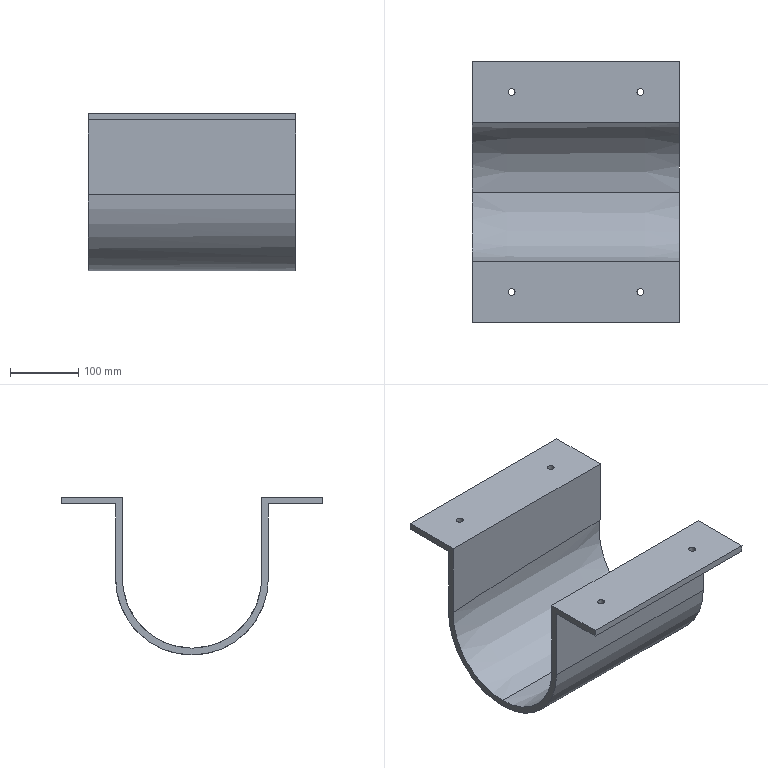Component | SolidWorks | Accessory1-3 | 1 solid | 31 faces | box 304.83 x 384.16 x 231.67 mm | volume 2139053 mm3 | plane 12 | cone 10 | cylinder 9 | commonest cylinder face diameters 10 x8 224.162 x1
STEP:
#1=COLOUR_RGB('',0.7922,0.8196,0.9333);
#2=FILL_AREA_STYLE_COLOUR('',#1);
#3=FILL_AREA_STYLE('',(#2));
#4=SURFACE_STYLE_FILL_AREA(#3);
#5=SURFACE_SIDE_STYLE('',(#4));
#6=SURFACE_STYLE_USAGE(.BOTH.,#5);
#7=PRESENTATION_STYLE_ASSIGNMENT((#6));
#8=CARTESIAN_POINT('',(-60.943,275.591,-4.023));
#9=VERTEX_POINT('',#8);
#10=CARTESIAN_POINT('',(-60.943,279.609,0.1806));
#11=VERTEX_POINT('',#10);
#12=CARTESIAN_POINT('',(-60.943,275.591,0.));
#13=DIRECTION('',(1.,-0.,-0.));
#14=DIRECTION('',(0.,0.,1.));
#15=AXIS2_PLACEMENT_3D('',#12,#13,#14);
#16=CIRCLE('',#15,4.023);
#17=EDGE_CURVE('',#9,#11,#16,.T.);
#18=ORIENTED_EDGE('',*,*,#17,.F.);
#19=CARTESIAN_POINT('',(-48.98,275.591,-4.088));
#20=VERTEX_POINT('',#19);
#21=CARTESIAN_POINT('',(-48.738,275.591,-4.089));
#22=DIRECTION('',(1.,-0.,-0.005413));
#23=VECTOR('',#22,39.37);
#24=LINE('',#21,#23);
#25=EDGE_CURVE('',#9,#20,#24,.T.);
#26=ORIENTED_EDGE('',*,*,#25,.T.);
#27=CARTESIAN_POINT('',(-48.959,279.609,0.7475));
#28=VERTEX_POINT('',#27);
#29=CARTESIAN_POINT('',(-48.98,275.591,-4.088));
#30=CARTESIAN_POINT('',(-48.98,278.35,-4.088));
#31=CARTESIAN_POINT('',(-48.971,280.114,-1.966));
#32=CARTESIAN_POINT('',(-48.959,279.609,0.7475));
#33=(BOUNDED_CURVE()B_SPLINE_CURVE(3,(#29,#30,#31,#32),.UNSPECIFIED.,.F.,.F.)B_SPLINE_CURVE_WITH_KNOTS((4,4),(3.142,4.896),.UNSPECIFIED.)CURVE()GEOMETRIC_REPRESENTATION_ITEM()RATIONAL_B_SPLINE_CURVE((1.,0.7595,0.7595,1.))REPRESENTATION_ITEM(''));
#34=EDGE_CURVE('',#20,#28,#33,.T.);
#35=ORIENTED_EDGE('',*,*,#34,.T.);
#36=CARTESIAN_POINT('',(-60.943,279.609,0.1806));
#37=CARTESIAN_POINT('',(-60.819,279.609,0.1956));
#38=CARTESIAN_POINT('',(-60.695,279.609,0.2088));
#39=CARTESIAN_POINT('',(-60.446,279.609,0.2333));
#40=CARTESIAN_POINT('',(-60.321,279.609,0.2446));
#41=CARTESIAN_POINT('',(-59.948,279.609,0.2765));
#42=CARTESIAN_POINT('',(-59.698,279.609,0.2953));
#43=CARTESIAN_POINT('',(-59.2,279.609,0.3301));
#44=CARTESIAN_POINT('',(-58.95,279.609,0.3461));
#45=CARTESIAN_POINT('',(-58.451,279.609,0.3763));
#46=CARTESIAN_POINT('',(-58.201,279.609,0.3904));
#47=CARTESIAN_POINT('',(-57.452,279.609,0.431));
#48=CARTESIAN_POINT('',(-56.953,279.609,0.4554));
#49=CARTESIAN_POINT('',(-55.954,279.609,0.5012));
#50=CARTESIAN_POINT('',(-55.455,279.609,0.5225));
#51=CARTESIAN_POINT('',(-53.956,279.609,0.5831));
#52=CARTESIAN_POINT('',(-52.957,279.609,0.6192));
#53=CARTESIAN_POINT('',(-50.958,279.609,0.6867));
#54=CARTESIAN_POINT('',(-49.958,279.609,0.7179));
#55=CARTESIAN_POINT('',(-48.959,279.609,0.7475));
#56=B_SPLINE_CURVE_WITH_KNOTS('',3,(#36,#37,#38,#39,#40,#41,#42,#43,#44,#45,#46,#47,#48,#49,#50,#51,#52,#53,#54,#55),.UNSPECIFIED.,.F.,.F.,(4,2,2,2,2,2,2,2,2,4),(0.02686,0.03643,0.046,0.06513,0.08427,0.1034,0.1417,0.18,0.2565,0.3331),.UNSPECIFIED.);
#57=EDGE_CURVE('',#11,#28,#56,.T.);
#58=ORIENTED_EDGE('',*,*,#57,.F.);
#59=EDGE_LOOP('',(#18,#26,#35,#58));
#60=FACE_OUTER_BOUND('',#59,.T.);
#61=CARTESIAN_POINT('',(-48.738,275.591,0.));
#62=DIRECTION('',(1.,-0.,-0.));
#63=DIRECTION('',(0.,0.,-1.));
#64=AXIS2_PLACEMENT_3D('',#61,#62,#63);
#65=CONICAL_SURFACE('',#64,4.089,0.005413);
#66=ADVANCED_FACE('',(#60),#65,.F.);
#67=CARTESIAN_POINT('',(-51.029,281.365,4.334));
#68=VERTEX_POINT('',#67);
#69=CARTESIAN_POINT('',(-51.422,281.365,4.334));
#70=VERTEX_POINT('',#69);
#71=CARTESIAN_POINT('',(-51.225,281.365,4.334));
#72=DIRECTION('',(-0.,0.,-1.));
#73=DIRECTION('',(-1.,0.,0.));
#74=AXIS2_PLACEMENT_3D('',#71,#72,#73);
#75=CIRCLE('',#74,0.1969);
#76=EDGE_CURVE('',#68,#70,#75,.T.);
#77=ORIENTED_EDGE('',*,*,#76,.F.);
#78=CARTESIAN_POINT('',(-51.009,281.365,4.315));
#79=VERTEX_POINT('',#78);
#80=CARTESIAN_POINT('',(-51.029,281.365,4.334));
#81=DIRECTION('',(0.7071,0.,-0.7071));
#82=VECTOR('',#81,39.37);
#83=LINE('',#80,#82);
#84=EDGE_CURVE('',#68,#79,#83,.T.);
#85=ORIENTED_EDGE('',*,*,#84,.T.);
#86=CARTESIAN_POINT('',(-51.442,281.365,4.315));
#87=VERTEX_POINT('',#86);
#88=CARTESIAN_POINT('',(-51.225,281.365,4.315));
#89=DIRECTION('',(0.,-0.,1.));
#90=DIRECTION('',(-1.,0.,0.));
#91=AXIS2_PLACEMENT_3D('',#88,#89,#90);
#92=CIRCLE('',#91,0.2165);
#93=EDGE_CURVE('',#87,#79,#92,.T.);
#94=ORIENTED_EDGE('',*,*,#93,.F.);
#95=CARTESIAN_POINT('',(-51.422,281.365,4.334));
#96=DIRECTION('',(-0.7071,0.,-0.7071));
#97=VECTOR('',#96,39.37);
#98=LINE('',#95,#97);
#99=EDGE_CURVE('',#70,#87,#98,.T.);
#100=ORIENTED_EDGE('',*,*,#99,.F.);
#101=EDGE_LOOP('',(#77,#85,#94,#100));
#102=FACE_OUTER_BOUND('',#101,.T.);
#103=CARTESIAN_POINT('',(-51.225,281.365,4.334));
#104=DIRECTION('',(-0.,0.,-1.));
#105=DIRECTION('',(-1.,0.,0.));
#106=AXIS2_PLACEMENT_3D('',#103,#104,#105);
#107=CONICAL_SURFACE('',#106,0.1969,0.7854);
#108=ADVANCED_FACE('',(#102),#107,.F.);
#109=CARTESIAN_POINT('',(-58.464,281.365,4.334));
#110=VERTEX_POINT('',#109);
#111=CARTESIAN_POINT('',(-58.858,281.365,4.334));
#112=VERTEX_POINT('',#111);
#113=CARTESIAN_POINT('',(-58.661,281.365,4.334));
#114=DIRECTION('',(-0.,0.,-1.));
#115=DIRECTION('',(-1.,0.,0.));
#116=AXIS2_PLACEMENT_3D('',#113,#114,#115);
#117=CIRCLE('',#116,0.1969);
#118=EDGE_CURVE('',#110,#112,#117,.T.);
#119=ORIENTED_EDGE('',*,*,#118,.F.);
#120=CARTESIAN_POINT('',(-58.445,281.365,4.315));
#121=VERTEX_POINT('',#120);
#122=CARTESIAN_POINT('',(-58.464,281.365,4.334));
#123=DIRECTION('',(0.7071,0.,-0.7071));
#124=VECTOR('',#123,39.37);
#125=LINE('',#122,#124);
#126=EDGE_CURVE('',#110,#121,#125,.T.);
#127=ORIENTED_EDGE('',*,*,#126,.T.);
#128=CARTESIAN_POINT('',(-58.878,281.365,4.315));
#129=VERTEX_POINT('',#128);
#130=CARTESIAN_POINT('',(-58.661,281.365,4.315));
#131=DIRECTION('',(0.,-0.,1.));
#132=DIRECTION('',(-1.,0.,0.));
#133=AXIS2_PLACEMENT_3D('',#130,#131,#132);
#134=CIRCLE('',#133,0.2165);
#135=EDGE_CURVE('',#129,#121,#134,.T.);
#136=ORIENTED_EDGE('',*,*,#135,.F.);
#137=CARTESIAN_POINT('',(-58.858,281.365,4.334));
#138=DIRECTION('',(-0.7071,0.,-0.7071));
#139=VECTOR('',#138,39.37);
#140=LINE('',#137,#139);
#141=EDGE_CURVE('',#112,#129,#140,.T.);
#142=ORIENTED_EDGE('',*,*,#141,.F.);
#143=EDGE_LOOP('',(#119,#127,#136,#142));
#144=FACE_OUTER_BOUND('',#143,.T.);
#145=CARTESIAN_POINT('',(-58.661,281.365,4.334));
#146=DIRECTION('',(-0.,0.,-1.));
#147=DIRECTION('',(-1.,0.,0.));
#148=AXIS2_PLACEMENT_3D('',#145,#146,#147);
#149=CONICAL_SURFACE('',#148,0.1969,0.7854);
#150=ADVANCED_FACE('',(#144),#149,.F.);
#151=CARTESIAN_POINT('',(-51.029,269.816,4.334));
#152=VERTEX_POINT('',#151);
#153=CARTESIAN_POINT('',(-51.422,269.816,4.334));
#154=VERTEX_POINT('',#153);
#155=CARTESIAN_POINT('',(-51.225,269.816,4.334));
#156=DIRECTION('',(-0.,0.,-1.));
#157=DIRECTION('',(-1.,0.,0.));
#158=AXIS2_PLACEMENT_3D('',#155,#156,#157);
#159=CIRCLE('',#158,0.1969);
#160=EDGE_CURVE('',#152,#154,#159,.T.);
#161=ORIENTED_EDGE('',*,*,#160,.F.);
#162=CARTESIAN_POINT('',(-51.009,269.816,4.315));
#163=VERTEX_POINT('',#162);
#164=CARTESIAN_POINT('',(-51.029,269.816,4.334));
#165=DIRECTION('',(0.7071,0.,-0.7071));
#166=VECTOR('',#165,39.37);
#167=LINE('',#164,#166);
#168=EDGE_CURVE('',#152,#163,#167,.T.);
#169=ORIENTED_EDGE('',*,*,#168,.T.);
#170=CARTESIAN_POINT('',(-51.442,269.816,4.315));
#171=VERTEX_POINT('',#170);
#172=CARTESIAN_POINT('',(-51.225,269.816,4.315));
#173=DIRECTION('',(0.,0.,1.));
#174=DIRECTION('',(0.,-1.,0.));
#175=AXIS2_PLACEMENT_3D('',#172,#173,#174);
#176=CIRCLE('',#175,0.2165);
#177=EDGE_CURVE('',#171,#163,#176,.T.);
#178=ORIENTED_EDGE('',*,*,#177,.F.);
#179=CARTESIAN_POINT('',(-51.422,269.816,4.334));
#180=DIRECTION('',(-0.7071,0.,-0.7071));
#181=VECTOR('',#180,39.37);
#182=LINE('',#179,#181);
#183=EDGE_CURVE('',#154,#171,#182,.T.);
#184=ORIENTED_EDGE('',*,*,#183,.F.);
#185=EDGE_LOOP('',(#161,#169,#178,#184));
#186=FACE_OUTER_BOUND('',#185,.T.);
#187=CARTESIAN_POINT('',(-51.225,269.816,4.334));
#188=DIRECTION('',(-0.,0.,-1.));
#189=DIRECTION('',(-1.,0.,0.));
#190=AXIS2_PLACEMENT_3D('',#187,#188,#189);
#191=CONICAL_SURFACE('',#190,0.1969,0.7854);
#192=ADVANCED_FACE('',(#186),#191,.F.);
#193=CARTESIAN_POINT('',(-58.464,269.816,4.334));
#194=VERTEX_POINT('',#193);
#195=CARTESIAN_POINT('',(-58.858,269.816,4.334));
#196=VERTEX_POINT('',#195);
#197=CARTESIAN_POINT('',(-58.661,269.816,4.334));
#198=DIRECTION('',(-0.,0.,-1.));
#199=DIRECTION('',(-1.,0.,0.));
#200=AXIS2_PLACEMENT_3D('',#197,#198,#199);
#201=CIRCLE('',#200,0.1969);
#202=EDGE_CURVE('',#194,#196,#201,.T.);
#203=ORIENTED_EDGE('',*,*,#202,.F.);
#204=CARTESIAN_POINT('',(-58.445,269.816,4.315));
#205=VERTEX_POINT('',#204);
#206=CARTESIAN_POINT('',(-58.464,269.816,4.334));
#207=DIRECTION('',(0.7071,0.,-0.7071));
#208=VECTOR('',#207,39.37);
#209=LINE('',#206,#208);
#210=EDGE_CURVE('',#194,#205,#209,.T.);
#211=ORIENTED_EDGE('',*,*,#210,.T.);
#212=CARTESIAN_POINT('',(-58.878,269.816,4.315));
#213=VERTEX_POINT('',#212);
#214=CARTESIAN_POINT('',(-58.661,269.816,4.315));
#215=DIRECTION('',(0.,0.,1.));
#216=DIRECTION('',(0.,-1.,0.));
#217=AXIS2_PLACEMENT_3D('',#214,#215,#216);
#218=CIRCLE('',#217,0.2165);
#219=EDGE_CURVE('',#213,#205,#218,.T.);
#220=ORIENTED_EDGE('',*,*,#219,.F.);
#221=CARTESIAN_POINT('',(-58.858,269.816,4.334));
#222=DIRECTION('',(-0.7071,0.,-0.7071));
#223=VECTOR('',#222,39.37);
#224=LINE('',#221,#223);
#225=EDGE_CURVE('',#196,#213,#224,.T.);
#226=ORIENTED_EDGE('',*,*,#225,.F.);
#227=EDGE_LOOP('',(#203,#211,#220,#226));
#228=FACE_OUTER_BOUND('',#227,.T.);
#229=CARTESIAN_POINT('',(-58.661,269.816,4.334));
#230=DIRECTION('',(-0.,0.,-1.));
#231=DIRECTION('',(-1.,0.,0.));
#232=AXIS2_PLACEMENT_3D('',#229,#230,#231);
#233=CONICAL_SURFACE('',#232,0.1969,0.7854);
#234=ADVANCED_FACE('',(#228),#233,.F.);
#235=CARTESIAN_POINT('',(-58.858,281.365,4.708));
#236=VERTEX_POINT('',#235);
#237=CARTESIAN_POINT('',(-58.464,281.365,4.708));
#238=VERTEX_POINT('',#237);
#239=CARTESIAN_POINT('',(-58.661,281.365,4.708));
#240=DIRECTION('',(0.,-0.,1.));
#241=DIRECTION('',(1.,0.,0.));
#242=AXIS2_PLACEMENT_3D('',#239,#240,#241);
#243=CIRCLE('',#242,0.1969);
#244=EDGE_CURVE('',#236,#238,#243,.T.);
#245=ORIENTED_EDGE('',*,*,#244,.T.);
#246=CARTESIAN_POINT('',(-58.464,281.365,18.882));
#247=DIRECTION('',(-0.,0.,-1.));
#248=VECTOR('',#247,39.37);
#249=LINE('',#246,#248);
#250=EDGE_CURVE('',#238,#110,#249,.T.);
#251=ORIENTED_EDGE('',*,*,#250,.T.);
#252=ORIENTED_EDGE('',*,*,#118,.T.);
#253=CARTESIAN_POINT('',(-58.858,281.365,18.882));
#254=DIRECTION('',(-0.,0.,-1.));
#255=VECTOR('',#254,39.37);
#256=LINE('',#253,#255);
#257=EDGE_CURVE('',#236,#112,#256,.T.);
#258=ORIENTED_EDGE('',*,*,#257,.F.);
#259=EDGE_LOOP('',(#245,#251,#252,#258));
#260=FACE_OUTER_BOUND('',#259,.T.);
#261=CARTESIAN_POINT('',(-58.661,281.365,18.882));
#262=DIRECTION('',(-0.,0.,-1.));
#263=DIRECTION('',(-1.,0.,0.));
#264=AXIS2_PLACEMENT_3D('',#261,#262,#263);
#265=CYLINDRICAL_SURFACE('',#264,0.1969);
#266=ADVANCED_FACE('',(#260),#265,.F.);
#267=CARTESIAN_POINT('',(-51.422,281.365,4.708));
#268=VERTEX_POINT('',#267);
#269=CARTESIAN_POINT('',(-51.029,281.365,4.708));
#270=VERTEX_POINT('',#269);
#271=CARTESIAN_POINT('',(-51.225,281.365,4.708));
#272=DIRECTION('',(0.,-0.,1.));
#273=DIRECTION('',(1.,0.,0.));
#274=AXIS2_PLACEMENT_3D('',#271,#272,#273);
#275=CIRCLE('',#274,0.1969);
#276=EDGE_CURVE('',#268,#270,#275,.T.);
#277=ORIENTED_EDGE('',*,*,#276,.T.);
#278=CARTESIAN_POINT('',(-51.029,281.365,18.882));
#279=DIRECTION('',(-0.,0.,-1.));
#280=VECTOR('',#279,39.37);
#281=LINE('',#278,#280);
#282=EDGE_CURVE('',#270,#68,#281,.T.);
#283=ORIENTED_EDGE('',*,*,#282,.T.);
#284=ORIENTED_EDGE('',*,*,#76,.T.);
#285=CARTESIAN_POINT('',(-51.422,281.365,18.882));
#286=DIRECTION('',(-0.,0.,-1.));
#287=VECTOR('',#286,39.37);
#288=LINE('',#285,#287);
#289=EDGE_CURVE('',#268,#70,#288,.T.);
#290=ORIENTED_EDGE('',*,*,#289,.F.);
#291=EDGE_LOOP('',(#277,#283,#284,#290));
#292=FACE_OUTER_BOUND('',#291,.T.);
#293=CARTESIAN_POINT('',(-51.225,281.365,18.882));
#294=DIRECTION('',(-0.,0.,-1.));
#295=DIRECTION('',(-1.,0.,0.));
#296=AXIS2_PLACEMENT_3D('',#293,#294,#295);
#297=CYLINDRICAL_SURFACE('',#296,0.1969);
#298=ADVANCED_FACE('',(#292),#297,.F.);
#299=CARTESIAN_POINT('',(-51.422,269.816,4.708));
#300=VERTEX_POINT('',#299);
#301=CARTESIAN_POINT('',(-51.029,269.816,4.708));
#302=VERTEX_POINT('',#301);
#303=CARTESIAN_POINT('',(-51.225,269.816,4.708));
#304=DIRECTION('',(0.,-0.,1.));
#305=DIRECTION('',(1.,0.,0.));
#306=AXIS2_PLACEMENT_3D('',#303,#304,#305);
#307=CIRCLE('',#306,0.1969);
#308=EDGE_CURVE('',#300,#302,#307,.T.);
#309=ORIENTED_EDGE('',*,*,#308,.T.);
#310=CARTESIAN_POINT('',(-51.029,269.816,18.882));
#311=DIRECTION('',(-0.,0.,-1.));
#312=VECTOR('',#311,39.37);
#313=LINE('',#310,#312);
#314=EDGE_CURVE('',#302,#152,#313,.T.);
#315=ORIENTED_EDGE('',*,*,#314,.T.);
#316=ORIENTED_EDGE('',*,*,#160,.T.);
#317=CARTESIAN_POINT('',(-51.422,269.816,18.882));
#318=DIRECTION('',(-0.,0.,-1.));
#319=VECTOR('',#318,39.37);
#320=LINE('',#317,#319);
#321=EDGE_CURVE('',#300,#154,#320,.T.);
#322=ORIENTED_EDGE('',*,*,#321,.F.);
#323=EDGE_LOOP('',(#309,#315,#316,#322));
#324=FACE_OUTER_BOUND('',#323,.T.);
#325=CARTESIAN_POINT('',(-51.225,269.816,18.882));
#326=DIRECTION('',(-0.,0.,-1.));
#327=DIRECTION('',(-1.,0.,0.));
#328=AXIS2_PLACEMENT_3D('',#325,#326,#327);
#329=CYLINDRICAL_SURFACE('',#328,0.1969);
#330=ADVANCED_FACE('',(#324),#329,.F.);
#331=CARTESIAN_POINT('',(-58.858,269.816,4.708));
#332=VERTEX_POINT('',#331);
#333=CARTESIAN_POINT('',(-58.464,269.816,4.708));
#334=VERTEX_POINT('',#333);
#335=CARTESIAN_POINT('',(-58.661,269.816,4.708));
#336=DIRECTION('',(0.,-0.,1.));
#337=DIRECTION('',(1.,0.,0.));
#338=AXIS2_PLACEMENT_3D('',#335,#336,#337);
#339=CIRCLE('',#338,0.1969);
#340=EDGE_CURVE('',#332,#334,#339,.T.);
#341=ORIENTED_EDGE('',*,*,#340,.T.);
#342=CARTESIAN_POINT('',(-58.464,269.816,18.882));
#343=DIRECTION('',(-0.,0.,-1.));
#344=VECTOR('',#343,39.37);
#345=LINE('',#342,#344);
#346=EDGE_CURVE('',#334,#194,#345,.T.);
#347=ORIENTED_EDGE('',*,*,#346,.T.);
#348=ORIENTED_EDGE('',*,*,#202,.T.);
#349=CARTESIAN_POINT('',(-58.858,269.816,18.882));
#350=DIRECTION('',(-0.,0.,-1.));
#351=VECTOR('',#350,39.37);
#352=LINE('',#349,#351);
#353=EDGE_CURVE('',#332,#196,#352,.T.);
#354=ORIENTED_EDGE('',*,*,#353,.F.);
#355=EDGE_LOOP('',(#341,#347,#348,#354));
#356=FACE_OUTER_BOUND('',#355,.T.);
#357=CARTESIAN_POINT('',(-58.661,269.816,18.882));
#358=DIRECTION('',(-0.,0.,-1.));
#359=DIRECTION('',(-1.,0.,0.));
#360=AXIS2_PLACEMENT_3D('',#357,#358,#359);
#361=CYLINDRICAL_SURFACE('',#360,0.1969);
#362=ADVANCED_FACE('',(#356),#361,.F.);
#363=CARTESIAN_POINT('',(-60.943,279.609,4.708));
#364=VERTEX_POINT('',#363);
#365=CARTESIAN_POINT('',(-60.943,279.609,0.));
#366=DIRECTION('',(0.,-0.,1.));
#367=VECTOR('',#366,39.37);
#368=LINE('',#365,#367);
#369=EDGE_CURVE('',#11,#364,#368,.T.);
#370=ORIENTED_EDGE('',*,*,#369,.F.);
#371=ORIENTED_EDGE('',*,*,#57,.T.);
#372=CARTESIAN_POINT('',(-48.942,279.609,4.708));
#373=VERTEX_POINT('',#372);
#374=CARTESIAN_POINT('',(-48.962,279.609,0.02033));
#375=DIRECTION('',(-0.004294,0.,-1.));
#376=VECTOR('',#375,39.37);
#377=LINE('',#374,#376);
#378=EDGE_CURVE('',#373,#28,#377,.T.);
#379=ORIENTED_EDGE('',*,*,#378,.F.);
#380=CARTESIAN_POINT('',(-44.227,279.609,4.708));
#381=DIRECTION('',(-1.,0.,0.));
#382=VECTOR('',#381,39.37);
#383=LINE('',#380,#382);
#384=EDGE_CURVE('',#373,#364,#383,.T.);
#385=ORIENTED_EDGE('',*,*,#384,.T.);
#386=EDGE_LOOP('',(#370,#371,#379,#385));
#387=FACE_OUTER_BOUND('',#386,.T.);
#388=CARTESIAN_POINT('',(-44.227,279.609,0.));
#389=DIRECTION('',(-0.,-1.,0.));
#390=DIRECTION('',(1.,-0.,-0.));
#391=AXIS2_PLACEMENT_3D('',#388,#389,#390);
#392=PLANE('',#391);
#393=ADVANCED_FACE('',(#387),#392,.T.);
#394=CARTESIAN_POINT('',(-48.959,271.572,0.7475));
#395=VERTEX_POINT('',#394);
#396=CARTESIAN_POINT('',(-48.942,271.572,4.708));
#397=VERTEX_POINT('',#396);
#398=CARTESIAN_POINT('',(-48.962,271.572,0.02033));
#399=DIRECTION('',(0.004294,-0.,1.));
#400=VECTOR('',#399,39.37);
#401=LINE('',#398,#400);
#402=EDGE_CURVE('',#395,#397,#401,.T.);
#403=ORIENTED_EDGE('',*,*,#402,.F.);
#404=CARTESIAN_POINT('',(-60.943,271.572,0.1806));
#405=VERTEX_POINT('',#404);
#406=CARTESIAN_POINT('',(-48.959,271.572,0.7475));
#407=CARTESIAN_POINT('',(-49.959,271.572,0.7179));
#408=CARTESIAN_POINT('',(-50.958,271.572,0.6867));
#409=CARTESIAN_POINT('',(-52.957,271.572,0.6192));
#410=CARTESIAN_POINT('',(-53.956,271.572,0.5831));
#411=CARTESIAN_POINT('',(-55.455,271.572,0.5224));
#412=CARTESIAN_POINT('',(-55.955,271.572,0.5011));
#413=CARTESIAN_POINT('',(-56.954,271.572,0.4554));
#414=CARTESIAN_POINT('',(-57.453,271.572,0.4309));
#415=CARTESIAN_POINT('',(-58.202,271.572,0.3904));
#416=CARTESIAN_POINT('',(-58.452,271.572,0.3762));
#417=CARTESIAN_POINT('',(-58.951,271.572,0.3461));
#418=CARTESIAN_POINT('',(-59.2,271.572,0.3301));
#419=CARTESIAN_POINT('',(-59.699,271.572,0.2953));
#420=CARTESIAN_POINT('',(-59.948,271.572,0.2765));
#421=CARTESIAN_POINT('',(-60.321,271.572,0.2446));
#422=CARTESIAN_POINT('',(-60.446,271.572,0.2333));
#423=CARTESIAN_POINT('',(-60.695,271.572,0.2088));
#424=CARTESIAN_POINT('',(-60.819,271.572,0.1956));
#425=CARTESIAN_POINT('',(-60.943,271.572,0.1806));
#426=B_SPLINE_CURVE_WITH_KNOTS('',3,(#406,#407,#408,#409,#410,#411,#412,#413,#414,#415,#416,#417,#418,#419,#420,#421,#422,#423,#424,#425),.UNSPECIFIED.,.F.,.F.,(4,2,2,2,2,2,2,2,2,4),(0.008057,0.08426,0.1605,0.1986,0.2367,0.2557,0.2748,0.2938,0.3033,0.3129),.UNSPECIFIED.);
#427=EDGE_CURVE('',#395,#405,#426,.T.);
#428=ORIENTED_EDGE('',*,*,#427,.T.);
#429=CARTESIAN_POINT('',(-60.943,271.572,4.708));
#430=VERTEX_POINT('',#429);
#431=CARTESIAN_POINT('',(-60.943,271.572,0.));
#432=DIRECTION('',(-0.,0.,-1.));
#433=VECTOR('',#432,39.37);
#434=LINE('',#431,#433);
#435=EDGE_CURVE('',#430,#405,#434,.T.);
#436=ORIENTED_EDGE('',*,*,#435,.F.);
#437=CARTESIAN_POINT('',(-44.227,271.572,4.708));
#438=DIRECTION('',(-1.,0.,0.));
#439=VECTOR('',#438,39.37);
#440=LINE('',#437,#439);
#441=EDGE_CURVE('',#397,#430,#440,.T.);
#442=ORIENTED_EDGE('',*,*,#441,.F.);
#443=EDGE_LOOP('',(#403,#428,#436,#442));
#444=FACE_OUTER_BOUND('',#443,.T.);
#445=CARTESIAN_POINT('',(-44.227,271.572,0.));
#446=DIRECTION('',(0.,1.,0.));
#447=DIRECTION('',(-1.,0.,0.));
#448=AXIS2_PLACEMENT_3D('',#445,#446,#447);
#449=PLANE('',#448);
#450=ADVANCED_FACE('',(#444),#449,.T.);
#451=CARTESIAN_POINT('',(-48.962,271.178,0.));
#452=VERTEX_POINT('',#451);
#453=CARTESIAN_POINT('',(-60.943,271.178,0.));
#454=VERTEX_POINT('',#453);
#455=CARTESIAN_POINT('',(-44.227,271.178,0.));
#456=DIRECTION('',(-1.,0.,0.));
#457=VECTOR('',#456,39.37);
#458=LINE('',#455,#457);
#459=EDGE_CURVE('',#452,#454,#458,.T.);
#460=ORIENTED_EDGE('',*,*,#459,.T.);
#461=CARTESIAN_POINT('',(-60.943,280.003,0.));
#462=VERTEX_POINT('',#461);
#463=CARTESIAN_POINT('',(-60.943,275.591,0.));
#464=DIRECTION('',(-1.,0.,0.));
#465=DIRECTION('',(0.,0.,1.));
#466=AXIS2_PLACEMENT_3D('',#463,#464,#465);
#467=CIRCLE('',#466,4.413);
#468=EDGE_CURVE('',#462,#454,#467,.T.);
#469=ORIENTED_EDGE('',*,*,#468,.F.);
#470=CARTESIAN_POINT('',(-48.962,280.003,0.));
#471=VERTEX_POINT('',#470);
#472=CARTESIAN_POINT('',(-44.227,280.003,0.));
#473=DIRECTION('',(-1.,0.,0.));
#474=VECTOR('',#473,39.37);
#475=LINE('',#472,#474);
#476=EDGE_CURVE('',#471,#462,#475,.T.);
#477=ORIENTED_EDGE('',*,*,#476,.F.);
#478=CARTESIAN_POINT('',(-48.962,271.178,0.));
#479=CARTESIAN_POINT('',(-49.,271.178,-8.825));
#480=CARTESIAN_POINT('',(-49.,280.003,-8.825));
#481=CARTESIAN_POINT('',(-48.962,280.003,0.));
#482=(BOUNDED_CURVE()B_SPLINE_CURVE(3,(#478,#479,#480,#481),.UNSPECIFIED.,.F.,.F.)B_SPLINE_CURVE_WITH_KNOTS((4,4),(4.712,7.854),.UNSPECIFIED.)CURVE()GEOMETRIC_REPRESENTATION_ITEM()RATIONAL_B_SPLINE_CURVE((1.,0.3333,0.3333,1.))REPRESENTATION_ITEM(''));
#483=EDGE_CURVE('',#452,#471,#482,.T.);
#484=ORIENTED_EDGE('',*,*,#483,.F.);
#485=EDGE_LOOP('',(#460,#469,#477,#484));
#486=FACE_OUTER_BOUND('',#485,.T.);
#487=CARTESIAN_POINT('',(-36.481,275.591,0.));
#488=DIRECTION('',(-1.,0.,0.));
#489=DIRECTION('',(0.,0.,1.));
#490=AXIS2_PLACEMENT_3D('',#487,#488,#489);
#491=CYLINDRICAL_SURFACE('',#490,4.413);
#492=ADVANCED_FACE('',(#486),#491,.T.);
#493=ORIENTED_EDGE('',*,*,#435,.T.);
#494=CARTESIAN_POINT('',(-60.943,275.591,0.));
#495=DIRECTION('',(1.,-0.,-0.));
#496=DIRECTION('',(0.,0.,1.));
#497=AXIS2_PLACEMENT_3D('',#494,#495,#496);
#498=CIRCLE('',#497,4.023);
#499=EDGE_CURVE('',#405,#9,#498,.T.);
#500=ORIENTED_EDGE('',*,*,#499,.T.);
#501=ORIENTED_EDGE('',*,*,#17,.T.);
#502=ORIENTED_EDGE('',*,*,#369,.T.);
#503=CARTESIAN_POINT('',(-60.943,283.153,4.708));
#504=VERTEX_POINT('',#503);
#505=CARTESIAN_POINT('',(-60.943,280.003,4.708));
#506=DIRECTION('',(0.,1.,0.));
#507=VECTOR('',#506,39.37);
#508=LINE('',#505,#507);
#509=EDGE_CURVE('',#364,#504,#508,.T.);
#510=ORIENTED_EDGE('',*,*,#509,.T.);
#511=CARTESIAN_POINT('',(-60.943,283.153,4.315));
#512=VERTEX_POINT('',#511);
#513=CARTESIAN_POINT('',(-60.943,283.153,4.708));
#514=DIRECTION('',(-0.,0.,-1.));
#515=VECTOR('',#514,39.37);
#516=LINE('',#513,#515);
#517=EDGE_CURVE('',#504,#512,#516,.T.);
#518=ORIENTED_EDGE('',*,*,#517,.T.);
#519=CARTESIAN_POINT('',(-60.943,280.003,4.315));
#520=VERTEX_POINT('',#519);
#521=CARTESIAN_POINT('',(-60.943,280.003,4.315));
#522=DIRECTION('',(-0.,-1.,0.));
#523=VECTOR('',#522,39.37);
#524=LINE('',#521,#523);
#525=EDGE_CURVE('',#512,#520,#524,.T.);
#526=ORIENTED_EDGE('',*,*,#525,.T.);
#527=CARTESIAN_POINT('',(-60.943,280.003,0.));
#528=DIRECTION('',(-0.,0.,-1.));
#529=VECTOR('',#528,39.37);
#530=LINE('',#527,#529);
#531=EDGE_CURVE('',#520,#462,#530,.T.);
#532=ORIENTED_EDGE('',*,*,#531,.T.);
#533=ORIENTED_EDGE('',*,*,#468,.T.);
#534=CARTESIAN_POINT('',(-60.943,271.178,4.315));
#535=VERTEX_POINT('',#534);
#536=CARTESIAN_POINT('',(-60.943,271.178,0.));
#537=DIRECTION('',(0.,-0.,1.));
#538=VECTOR('',#537,39.37);
#539=LINE('',#536,#538);
#540=EDGE_CURVE('',#454,#535,#539,.T.);
#541=ORIENTED_EDGE('',*,*,#540,.T.);
#542=CARTESIAN_POINT('',(-60.943,268.028,4.315));
#543=VERTEX_POINT('',#542);
#544=CARTESIAN_POINT('',(-60.943,271.178,4.315));
#545=DIRECTION('',(-0.,-1.,0.));
#546=VECTOR('',#545,39.37);
#547=LINE('',#544,#546);
#548=EDGE_CURVE('',#535,#543,#547,.T.);
#549=ORIENTED_EDGE('',*,*,#548,.T.);
#550=CARTESIAN_POINT('',(-60.943,268.028,4.708));
#551=VERTEX_POINT('',#550);
#552=CARTESIAN_POINT('',(-60.943,268.028,4.708));
#553=DIRECTION('',(0.,-0.,1.));
#554=VECTOR('',#553,39.37);
#555=LINE('',#552,#554);
#556=EDGE_CURVE('',#543,#551,#555,.T.);
#557=ORIENTED_EDGE('',*,*,#556,.T.);
#558=CARTESIAN_POINT('',(-60.943,271.572,4.708));
#559=DIRECTION('',(0.,1.,0.));
#560=VECTOR('',#559,39.37);
#561=LINE('',#558,#560);
#562=EDGE_CURVE('',#551,#430,#561,.T.);
#563=ORIENTED_EDGE('',*,*,#562,.T.);
#564=EDGE_LOOP('',(#493,#500,#501,#502,#510,#518,#526,#532,#533,#541,#549,#557,#563));
#565=FACE_OUTER_BOUND('',#564,.T.);
#566=CARTESIAN_POINT('',(-60.943,275.591,0.));
#567=DIRECTION('',(-1.,0.,0.));
#568=DIRECTION('',(0.,-0.,1.));
#569=AXIS2_PLACEMENT_3D('',#566,#567,#568);
#570=PLANE('',#569);
#571=ADVANCED_FACE('',(#565),#570,.T.);
#572=CARTESIAN_POINT('',(-48.959,271.572,0.7475));
#573=CARTESIAN_POINT('',(-48.971,271.067,-1.966));
#574=CARTESIAN_POINT('',(-48.98,272.831,-4.088));
#575=CARTESIAN_POINT('',(-48.98,275.591,-4.088));
#576=(BOUNDED_CURVE()B_SPLINE_CURVE(3,(#572,#573,#574,#575),.UNSPECIFIED.,.F.,.T.)B_SPLINE_CURVE_WITH_KNOTS((4,4),(1.387,3.142),.UNSPECIFIED.)CURVE()GEOMETRIC_REPRESENTATION_ITEM()RATIONAL_B_SPLINE_CURVE((1.,0.7595,0.7595,1.))REPRESENTATION_ITEM(''));
#577=EDGE_CURVE('',#395,#20,#576,.T.);
#578=ORIENTED_EDGE('',*,*,#577,.F.);
#579=ORIENTED_EDGE('',*,*,#402,.T.);
#580=CARTESIAN_POINT('',(-48.942,268.028,4.708));
#581=VERTEX_POINT('',#580);
#582=CARTESIAN_POINT('',(-48.942,271.572,4.708));
#583=DIRECTION('',(-0.,-1.,0.));
#584=VECTOR('',#583,39.37);
#585=LINE('',#582,#584);
#586=EDGE_CURVE('',#397,#581,#585,.T.);
#587=ORIENTED_EDGE('',*,*,#586,.T.);
#588=CARTESIAN_POINT('',(-48.944,268.028,4.315));
#589=VERTEX_POINT('',#588);
#590=CARTESIAN_POINT('',(-48.942,268.028,4.722));
#591=DIRECTION('',(-0.004294,0.,-1.));
#592=VECTOR('',#591,39.37);
#593=LINE('',#590,#592);
#594=EDGE_CURVE('',#581,#589,#593,.T.);
#595=ORIENTED_EDGE('',*,*,#594,.T.);
#596=CARTESIAN_POINT('',(-48.944,271.178,4.315));
#597=VERTEX_POINT('',#596);
#598=CARTESIAN_POINT('',(-48.944,271.178,4.315));
#599=DIRECTION('',(0.,1.,-0.));
#600=VECTOR('',#599,39.37);
#601=LINE('',#598,#600);
#602=EDGE_CURVE('',#589,#597,#601,.T.);
#603=ORIENTED_EDGE('',*,*,#602,.T.);
#604=CARTESIAN_POINT('',(-48.962,271.178,0.02033));
#605=DIRECTION('',(-0.004294,0.,-1.));
#606=VECTOR('',#605,39.37);
#607=LINE('',#604,#606);
#608=EDGE_CURVE('',#597,#452,#607,.T.);
#609=ORIENTED_EDGE('',*,*,#608,.T.);
#610=ORIENTED_EDGE('',*,*,#483,.T.);
#611=CARTESIAN_POINT('',(-48.944,280.003,4.315));
#612=VERTEX_POINT('',#611);
#613=CARTESIAN_POINT('',(-48.962,280.003,0.02033));
#614=DIRECTION('',(0.004294,-0.,1.));
#615=VECTOR('',#614,39.37);
#616=LINE('',#613,#615);
#617=EDGE_CURVE('',#471,#612,#616,.T.);
#618=ORIENTED_EDGE('',*,*,#617,.T.);
#619=CARTESIAN_POINT('',(-48.944,283.153,4.315));
#620=VERTEX_POINT('',#619);
#621=CARTESIAN_POINT('',(-48.944,280.003,4.315));
#622=DIRECTION('',(0.,1.,-0.));
#623=VECTOR('',#622,39.37);
#624=LINE('',#621,#623);
#625=EDGE_CURVE('',#612,#620,#624,.T.);
#626=ORIENTED_EDGE('',*,*,#625,.T.);
#627=CARTESIAN_POINT('',(-48.942,283.153,4.708));
#628=VERTEX_POINT('',#627);
#629=CARTESIAN_POINT('',(-48.942,283.153,4.722));
#630=DIRECTION('',(0.004294,-0.,1.));
#631=VECTOR('',#630,39.37);
#632=LINE('',#629,#631);
#633=EDGE_CURVE('',#620,#628,#632,.T.);
#634=ORIENTED_EDGE('',*,*,#633,.T.);
#635=CARTESIAN_POINT('',(-48.942,280.003,4.708));
#636=DIRECTION('',(-0.,-1.,0.));
#637=VECTOR('',#636,39.37);
#638=LINE('',#635,#637);
#639=EDGE_CURVE('',#628,#373,#638,.T.);
#640=ORIENTED_EDGE('',*,*,#639,.T.);
#641=ORIENTED_EDGE('',*,*,#378,.T.);
#642=ORIENTED_EDGE('',*,*,#34,.F.);
#643=EDGE_LOOP('',(#578,#579,#587,#595,#603,#609,#610,#618,#626,#634,#640,#641,#642));
#644=FACE_OUTER_BOUND('',#643,.T.);
#645=CARTESIAN_POINT('',(-48.902,290.564,14.07));
#646=DIRECTION('',(-1.,0.,0.004294));
#647=DIRECTION('',(-0.004294,-0.,-1.));
#648=AXIS2_PLACEMENT_3D('',#645,#646,#647);
#649=PLANE('',#648);
#650=ADVANCED_FACE('',(#644),#649,.F.);
#651=CARTESIAN_POINT('',(-45.769,280.003,4.315));
#652=DIRECTION('',(-1.,0.,0.));
#653=VECTOR('',#652,39.37);
#654=LINE('',#651,#653);
#655=EDGE_CURVE('',#612,#520,#654,.T.);
#656=ORIENTED_EDGE('',*,*,#655,.F.);
#657=ORIENTED_EDGE('',*,*,#617,.F.);
#658=ORIENTED_EDGE('',*,*,#476,.T.);
#659=ORIENTED_EDGE('',*,*,#531,.F.);
#660=EDGE_LOOP('',(#656,#657,#658,#659));
#661=FACE_OUTER_BOUND('',#660,.T.);
#662=CARTESIAN_POINT('',(-44.227,280.003,0.));
#663=DIRECTION('',(0.,1.,0.));
#664=DIRECTION('',(-1.,0.,0.));
#665=AXIS2_PLACEMENT_3D('',#662,#663,#664);
#666=PLANE('',#665);
#667=ADVANCED_FACE('',(#661),#666,.T.);
#668=ORIENTED_EDGE('',*,*,#244,.F.);
#669=CARTESIAN_POINT('',(-58.661,281.365,4.708));
#670=DIRECTION('',(0.,-0.,1.));
#671=DIRECTION('',(1.,0.,0.));
#672=AXIS2_PLACEMENT_3D('',#669,#670,#671);
#673=CIRCLE('',#672,0.1969);
#674=EDGE_CURVE('',#238,#236,#673,.T.);
#675=ORIENTED_EDGE('',*,*,#674,.F.);
#676=EDGE_LOOP('',(#668,#675));
#677=FACE_BOUND('',#676,.T.);
#678=ORIENTED_EDGE('',*,*,#276,.F.);
#679=CARTESIAN_POINT('',(-51.225,281.365,4.708));
#680=DIRECTION('',(0.,-0.,1.));
#681=DIRECTION('',(1.,0.,0.));
#682=AXIS2_PLACEMENT_3D('',#679,#680,#681);
#683=CIRCLE('',#682,0.1969);
#684=EDGE_CURVE('',#270,#268,#683,.T.);
#685=ORIENTED_EDGE('',*,*,#684,.F.);
#686=EDGE_LOOP('',(#678,#685));
#687=FACE_BOUND('',#686,.T.);
#688=ORIENTED_EDGE('',*,*,#639,.F.);
#689=CARTESIAN_POINT('',(-45.769,283.153,4.708));
#690=DIRECTION('',(-1.,0.,0.));
#691=VECTOR('',#690,39.37);
#692=LINE('',#689,#691);
#693=EDGE_CURVE('',#628,#504,#692,.T.);
#694=ORIENTED_EDGE('',*,*,#693,.T.);
#695=ORIENTED_EDGE('',*,*,#509,.F.);
#696=ORIENTED_EDGE('',*,*,#384,.F.);
#697=EDGE_LOOP('',(#688,#694,#695,#696));
#698=FACE_OUTER_BOUND('',#697,.T.);
#699=CARTESIAN_POINT('',(-44.227,280.003,4.708));
#700=DIRECTION('',(0.,-0.,1.));
#701=DIRECTION('',(1.,-0.,-0.));
#702=AXIS2_PLACEMENT_3D('',#699,#700,#701);
#703=PLANE('',#702);
#704=ADVANCED_FACE('',(#677,#687,#698),#703,.T.);
#705=ORIENTED_EDGE('',*,*,#308,.F.);
#706=CARTESIAN_POINT('',(-51.225,269.816,4.708));
#707=DIRECTION('',(0.,-0.,1.));
#708=DIRECTION('',(1.,0.,0.));
#709=AXIS2_PLACEMENT_3D('',#706,#707,#708);
#710=CIRCLE('',#709,0.1969);
#711=EDGE_CURVE('',#302,#300,#710,.T.);
#712=ORIENTED_EDGE('',*,*,#711,.F.);
#713=EDGE_LOOP('',(#705,#712));
#714=FACE_BOUND('',#713,.T.);
#715=ORIENTED_EDGE('',*,*,#340,.F.);
#716=CARTESIAN_POINT('',(-58.661,269.816,4.708));
#717=DIRECTION('',(0.,-0.,1.));
#718=DIRECTION('',(1.,0.,0.));
#719=AXIS2_PLACEMENT_3D('',#716,#717,#718);
#720=CIRCLE('',#719,0.1969);
#721=EDGE_CURVE('',#334,#332,#720,.T.);
#722=ORIENTED_EDGE('',*,*,#721,.F.);
#723=EDGE_LOOP('',(#715,#722));
#724=FACE_BOUND('',#723,.T.);
#725=ORIENTED_EDGE('',*,*,#586,.F.);
#726=ORIENTED_EDGE('',*,*,#441,.T.);
#727=ORIENTED_EDGE('',*,*,#562,.F.);
#728=CARTESIAN_POINT('',(-45.769,268.028,4.708));
#729=DIRECTION('',(-1.,0.,0.));
#730=VECTOR('',#729,39.37);
#731=LINE('',#728,#730);
#732=EDGE_CURVE('',#581,#551,#731,.T.);
#733=ORIENTED_EDGE('',*,*,#732,.F.);
#734=EDGE_LOOP('',(#725,#726,#727,#733));
#735=FACE_OUTER_BOUND('',#734,.T.);
#736=CARTESIAN_POINT('',(-44.227,271.572,4.708));
#737=DIRECTION('',(0.,-0.,1.));
#738=DIRECTION('',(1.,-0.,-0.));
#739=AXIS2_PLACEMENT_3D('',#736,#737,#738);
#740=PLANE('',#739);
#741=ADVANCED_FACE('',(#714,#724,#735),#740,.T.);
#742=CARTESIAN_POINT('',(-45.769,271.178,4.315));
#743=DIRECTION('',(-1.,0.,0.));
#744=VECTOR('',#743,39.37);
#745=LINE('',#742,#744);
#746=EDGE_CURVE('',#597,#535,#745,.T.);
#747=ORIENTED_EDGE('',*,*,#746,.T.);
#748=ORIENTED_EDGE('',*,*,#540,.F.);
#749=ORIENTED_EDGE('',*,*,#459,.F.);
#750=ORIENTED_EDGE('',*,*,#608,.F.);
#751=EDGE_LOOP('',(#747,#748,#749,#750));
#752=FACE_OUTER_BOUND('',#751,.T.);
#753=CARTESIAN_POINT('',(-44.227,271.178,0.));
#754=DIRECTION('',(-0.,-1.,0.));
#755=DIRECTION('',(1.,-0.,-0.));
#756=AXIS2_PLACEMENT_3D('',#753,#754,#755);
#757=PLANE('',#756);
#758=ADVANCED_FACE('',(#752),#757,.T.);
#759=ORIENTED_EDGE('',*,*,#135,.T.);
#760=CARTESIAN_POINT('',(-58.661,281.365,4.315));
#761=DIRECTION('',(0.,-0.,1.));
#762=DIRECTION('',(-1.,0.,0.));
#763=AXIS2_PLACEMENT_3D('',#760,#761,#762);
#764=CIRCLE('',#763,0.2165);
#765=EDGE_CURVE('',#121,#129,#764,.T.);
#766=ORIENTED_EDGE('',*,*,#765,.T.);
#767=EDGE_LOOP('',(#759,#766));
#768=FACE_BOUND('',#767,.T.);
#769=ORIENTED_EDGE('',*,*,#93,.T.);
#770=CARTESIAN_POINT('',(-51.225,281.365,4.315));
#771=DIRECTION('',(0.,-0.,1.));
#772=DIRECTION('',(-1.,0.,0.));
#773=AXIS2_PLACEMENT_3D('',#770,#771,#772);
#774=CIRCLE('',#773,0.2165);
#775=EDGE_CURVE('',#79,#87,#774,.T.);
#776=ORIENTED_EDGE('',*,*,#775,.T.);
#777=EDGE_LOOP('',(#769,#776));
#778=FACE_BOUND('',#777,.T.);
#779=ORIENTED_EDGE('',*,*,#625,.F.);
#780=ORIENTED_EDGE('',*,*,#655,.T.);
#781=ORIENTED_EDGE('',*,*,#525,.F.);
#782=CARTESIAN_POINT('',(-45.769,283.153,4.315));
#783=DIRECTION('',(-1.,0.,0.));
#784=VECTOR('',#783,39.37);
#785=LINE('',#782,#784);
#786=EDGE_CURVE('',#620,#512,#785,.T.);
#787=ORIENTED_EDGE('',*,*,#786,.F.);
#788=EDGE_LOOP('',(#779,#780,#781,#787));
#789=FACE_OUTER_BOUND('',#788,.T.);
#790=CARTESIAN_POINT('',(-45.769,280.003,4.315));
#791=DIRECTION('',(-0.,0.,-1.));
#792=DIRECTION('',(-1.,0.,0.));
#793=AXIS2_PLACEMENT_3D('',#790,#791,#792);
#794=PLANE('',#793);
#795=ADVANCED_FACE('',(#768,#778,#789),#794,.T.);
#796=ORIENTED_EDGE('',*,*,#633,.F.);
#797=ORIENTED_EDGE('',*,*,#786,.T.);
#798=ORIENTED_EDGE('',*,*,#517,.F.);
#799=ORIENTED_EDGE('',*,*,#693,.F.);
#800=EDGE_LOOP('',(#796,#797,#798,#799));
#801=FACE_OUTER_BOUND('',#800,.T.);
#802=CARTESIAN_POINT('',(-45.769,283.153,4.708));
#803=DIRECTION('',(0.,1.,0.));
#804=DIRECTION('',(-1.,0.,0.));
#805=AXIS2_PLACEMENT_3D('',#802,#803,#804);
#806=PLANE('',#805);
#807=ADVANCED_FACE('',(#801),#806,.T.);
#808=ORIENTED_EDGE('',*,*,#594,.F.);
#809=ORIENTED_EDGE('',*,*,#732,.T.);
#810=ORIENTED_EDGE('',*,*,#556,.F.);
#811=CARTESIAN_POINT('',(-45.769,268.028,4.315));
#812=DIRECTION('',(-1.,0.,0.));
#813=VECTOR('',#812,39.37);
#814=LINE('',#811,#813);
#815=EDGE_CURVE('',#589,#543,#814,.T.);
#816=ORIENTED_EDGE('',*,*,#815,.F.);
#817=EDGE_LOOP('',(#808,#809,#810,#816));
#818=FACE_OUTER_BOUND('',#817,.T.);
#819=CARTESIAN_POINT('',(-45.769,268.028,4.708));
#820=DIRECTION('',(-0.,-1.,0.));
#821=DIRECTION('',(1.,-0.,-0.));
#822=AXIS2_PLACEMENT_3D('',#819,#820,#821);
#823=PLANE('',#822);
#824=ADVANCED_FACE('',(#818),#823,.T.);
#825=ORIENTED_EDGE('',*,*,#219,.T.);
#826=CARTESIAN_POINT('',(-58.661,269.816,4.315));
#827=DIRECTION('',(0.,0.,1.));
#828=DIRECTION('',(0.,-1.,0.));
#829=AXIS2_PLACEMENT_3D('',#826,#827,#828);
#830=CIRCLE('',#829,0.2165);
#831=EDGE_CURVE('',#205,#213,#830,.T.);
#832=ORIENTED_EDGE('',*,*,#831,.T.);
#833=EDGE_LOOP('',(#825,#832));
#834=FACE_BOUND('',#833,.T.);
#835=ORIENTED_EDGE('',*,*,#177,.T.);
#836=CARTESIAN_POINT('',(-51.225,269.816,4.315));
#837=DIRECTION('',(0.,0.,1.));
#838=DIRECTION('',(0.,-1.,0.));
#839=AXIS2_PLACEMENT_3D('',#836,#837,#838);
#840=CIRCLE('',#839,0.2165);
#841=EDGE_CURVE('',#163,#171,#840,.T.);
#842=ORIENTED_EDGE('',*,*,#841,.T.);
#843=EDGE_LOOP('',(#835,#842));
#844=FACE_BOUND('',#843,.T.);
#845=ORIENTED_EDGE('',*,*,#602,.F.);
#846=ORIENTED_EDGE('',*,*,#815,.T.);
#847=ORIENTED_EDGE('',*,*,#548,.F.);
#848=ORIENTED_EDGE('',*,*,#746,.F.);
#849=EDGE_LOOP('',(#845,#846,#847,#848));
#850=FACE_OUTER_BOUND('',#849,.T.);
#851=CARTESIAN_POINT('',(-45.769,271.178,4.315));
#852=DIRECTION('',(-0.,-0.,-1.));
#853=DIRECTION('',(-0.,-1.,0.));
#854=AXIS2_PLACEMENT_3D('',#851,#852,#853);
#855=PLANE('',#854);
#856=ADVANCED_FACE('',(#834,#844,#850),#855,.T.);
#857=ORIENTED_EDGE('',*,*,#346,.F.);
#858=ORIENTED_EDGE('',*,*,#721,.T.);
#859=ORIENTED_EDGE('',*,*,#353,.T.);
#860=CARTESIAN_POINT('',(-58.661,269.816,4.334));
#861=DIRECTION('',(-0.,0.,-1.));
#862=DIRECTION('',(-1.,0.,0.));
#863=AXIS2_PLACEMENT_3D('',#860,#861,#862);
#864=CIRCLE('',#863,0.1969);
#865=EDGE_CURVE('',#196,#194,#864,.T.);
#866=ORIENTED_EDGE('',*,*,#865,.T.);
#867=EDGE_LOOP('',(#857,#858,#859,#866));
#868=FACE_OUTER_BOUND('',#867,.T.);
#869=CARTESIAN_POINT('',(-58.661,269.816,18.882));
#870=DIRECTION('',(-0.,0.,-1.));
#871=DIRECTION('',(-1.,0.,0.));
#872=AXIS2_PLACEMENT_3D('',#869,#870,#871);
#873=CYLINDRICAL_SURFACE('',#872,0.1969);
#874=ADVANCED_FACE('',(#868),#873,.F.);
#875=ORIENTED_EDGE('',*,*,#314,.F.);
#876=ORIENTED_EDGE('',*,*,#711,.T.);
#877=ORIENTED_EDGE('',*,*,#321,.T.);
#878=CARTESIAN_POINT('',(-51.225,269.816,4.334));
#879=DIRECTION('',(-0.,0.,-1.));
#880=DIRECTION('',(-1.,0.,0.));
#881=AXIS2_PLACEMENT_3D('',#878,#879,#880);
#882=CIRCLE('',#881,0.1969);
#883=EDGE_CURVE('',#154,#152,#882,.T.);
#884=ORIENTED_EDGE('',*,*,#883,.T.);
#885=EDGE_LOOP('',(#875,#876,#877,#884));
#886=FACE_OUTER_BOUND('',#885,.T.);
#887=CARTESIAN_POINT('',(-51.225,269.816,18.882));
#888=DIRECTION('',(-0.,0.,-1.));
#889=DIRECTION('',(-1.,0.,0.));
#890=AXIS2_PLACEMENT_3D('',#887,#888,#889);
#891=CYLINDRICAL_SURFACE('',#890,0.1969);
#892=ADVANCED_FACE('',(#886),#891,.F.);
#893=ORIENTED_EDGE('',*,*,#282,.F.);
#894=ORIENTED_EDGE('',*,*,#684,.T.);
#895=ORIENTED_EDGE('',*,*,#289,.T.);
#896=CARTESIAN_POINT('',(-51.225,281.365,4.334));
#897=DIRECTION('',(-0.,0.,-1.));
#898=DIRECTION('',(-1.,0.,0.));
#899=AXIS2_PLACEMENT_3D('',#896,#897,#898);
#900=CIRCLE('',#899,0.1969);
#901=EDGE_CURVE('',#70,#68,#900,.T.);
#902=ORIENTED_EDGE('',*,*,#901,.T.);
#903=EDGE_LOOP('',(#893,#894,#895,#902));
#904=FACE_OUTER_BOUND('',#903,.T.);
#905=CARTESIAN_POINT('',(-51.225,281.365,18.882));
#906=DIRECTION('',(-0.,0.,-1.));
#907=DIRECTION('',(-1.,0.,0.));
#908=AXIS2_PLACEMENT_3D('',#905,#906,#907);
#909=CYLINDRICAL_SURFACE('',#908,0.1969);
#910=ADVANCED_FACE('',(#904),#909,.F.);
#911=ORIENTED_EDGE('',*,*,#250,.F.);
#912=ORIENTED_EDGE('',*,*,#674,.T.);
#913=ORIENTED_EDGE('',*,*,#257,.T.);
#914=CARTESIAN_POINT('',(-58.661,281.365,4.334));
#915=DIRECTION('',(-0.,0.,-1.));
#916=DIRECTION('',(-1.,0.,0.));
#917=AXIS2_PLACEMENT_3D('',#914,#915,#916);
#918=CIRCLE('',#917,0.1969);
#919=EDGE_CURVE('',#112,#110,#918,.T.);
#920=ORIENTED_EDGE('',*,*,#919,.T.);
#921=EDGE_LOOP('',(#911,#912,#913,#920));
#922=FACE_OUTER_BOUND('',#921,.T.);
#923=CARTESIAN_POINT('',(-58.661,281.365,18.882));
#924=DIRECTION('',(-0.,0.,-1.));
#925=DIRECTION('',(-1.,0.,0.));
#926=AXIS2_PLACEMENT_3D('',#923,#924,#925);
#927=CYLINDRICAL_SURFACE('',#926,0.1969);
#928=ADVANCED_FACE('',(#922),#927,.F.);
#929=ORIENTED_EDGE('',*,*,#210,.F.);
#930=ORIENTED_EDGE('',*,*,#865,.F.);
#931=ORIENTED_EDGE('',*,*,#225,.T.);
#932=ORIENTED_EDGE('',*,*,#831,.F.);
#933=EDGE_LOOP('',(#929,#930,#931,#932));
#934=FACE_OUTER_BOUND('',#933,.T.);
#935=CARTESIAN_POINT('',(-58.661,269.816,4.334));
#936=DIRECTION('',(-0.,0.,-1.));
#937=DIRECTION('',(-1.,0.,0.));
#938=AXIS2_PLACEMENT_3D('',#935,#936,#937);
#939=CONICAL_SURFACE('',#938,0.1969,0.7854);
#940=ADVANCED_FACE('',(#934),#939,.F.);
#941=ORIENTED_EDGE('',*,*,#168,.F.);
#942=ORIENTED_EDGE('',*,*,#883,.F.);
#943=ORIENTED_EDGE('',*,*,#183,.T.);
#944=ORIENTED_EDGE('',*,*,#841,.F.);
#945=EDGE_LOOP('',(#941,#942,#943,#944));
#946=FACE_OUTER_BOUND('',#945,.T.);
#947=CARTESIAN_POINT('',(-51.225,269.816,4.334));
#948=DIRECTION('',(-0.,0.,-1.));
#949=DIRECTION('',(-1.,0.,0.));
#950=AXIS2_PLACEMENT_3D('',#947,#948,#949);
#951=CONICAL_SURFACE('',#950,0.1969,0.7854);
#952=ADVANCED_FACE('',(#946),#951,.F.);
#953=ORIENTED_EDGE('',*,*,#126,.F.);
#954=ORIENTED_EDGE('',*,*,#919,.F.);
#955=ORIENTED_EDGE('',*,*,#141,.T.);
#956=ORIENTED_EDGE('',*,*,#765,.F.);
#957=EDGE_LOOP('',(#953,#954,#955,#956));
#958=FACE_OUTER_BOUND('',#957,.T.);
#959=CARTESIAN_POINT('',(-58.661,281.365,4.334));
#960=DIRECTION('',(-0.,0.,-1.));
#961=DIRECTION('',(-1.,0.,0.));
#962=AXIS2_PLACEMENT_3D('',#959,#960,#961);
#963=CONICAL_SURFACE('',#962,0.1969,0.7854);
#964=ADVANCED_FACE('',(#958),#963,.F.);
#965=ORIENTED_EDGE('',*,*,#84,.F.);
#966=ORIENTED_EDGE('',*,*,#901,.F.);
#967=ORIENTED_EDGE('',*,*,#99,.T.);
#968=ORIENTED_EDGE('',*,*,#775,.F.);
#969=EDGE_LOOP('',(#965,#966,#967,#968));
#970=FACE_OUTER_BOUND('',#969,.T.);
#971=CARTESIAN_POINT('',(-51.225,281.365,4.334));
#972=DIRECTION('',(-0.,0.,-1.));
#973=DIRECTION('',(-1.,0.,0.));
#974=AXIS2_PLACEMENT_3D('',#971,#972,#973);
#975=CONICAL_SURFACE('',#974,0.1969,0.7854);
#976=ADVANCED_FACE('',(#970),#975,.F.);
#977=ORIENTED_EDGE('',*,*,#25,.F.);
#978=ORIENTED_EDGE('',*,*,#499,.F.);
#979=ORIENTED_EDGE('',*,*,#427,.F.);
#980=ORIENTED_EDGE('',*,*,#577,.T.);
#981=EDGE_LOOP('',(#977,#978,#979,#980));
#982=FACE_OUTER_BOUND('',#981,.T.);
#983=CARTESIAN_POINT('',(-48.738,275.591,0.));
#984=DIRECTION('',(1.,-0.,-0.));
#985=DIRECTION('',(0.,0.,-1.));
#986=AXIS2_PLACEMENT_3D('',#983,#984,#985);
#987=CONICAL_SURFACE('',#986,4.089,0.005413);
#988=ADVANCED_FACE('',(#982),#987,.F.);
#989=CLOSED_SHELL('',(#66,#108,#150,#192,#234,#266,#298,#330,#362,#393,#450,#492,#571,#650,#667,#704,#741,#758,#795,#807,#824,#856,#874,#892,#910,#928,#940,#952,#964,#976,#988));
#990=MANIFOLD_SOLID_BREP('',#989);
#991=STYLED_ITEM('',(#7),#990);
#992=PRESENTATION_LAYER_ASSIGNMENT('','',(#991));
#993=CARTESIAN_POINT('',(0.,0.,0.));
#994=DIRECTION('',(0.,0.,1.));
#995=DIRECTION('',(1.,0.,0.));
#996=AXIS2_PLACEMENT_3D('',#993,#994,#995);
#997=(LENGTH_UNIT()NAMED_UNIT(*)SI_UNIT($,.METRE.));
#998=LENGTH_MEASURE_WITH_UNIT(LENGTH_MEASURE(0.0254),#997);
#999=DIMENSIONAL_EXPONENTS(1.,0.,0.,0.,0.,0.,0.);
#1000=(CONVERSION_BASED_UNIT('',#998)LENGTH_UNIT()NAMED_UNIT(#999));
#1001=UNCERTAINTY_MEASURE_WITH_UNIT(LENGTH_MEASURE(0.00001),#1000,'','');
#1002=(NAMED_UNIT(*)PLANE_ANGLE_UNIT()SI_UNIT($,.RADIAN.));
#1003=(NAMED_UNIT(*)SI_UNIT($,.STERADIAN.)SOLID_ANGLE_UNIT());
#1004=(GEOMETRIC_REPRESENTATION_CONTEXT(3)GLOBAL_UNCERTAINTY_ASSIGNED_CONTEXT((#1001))GLOBAL_UNIT_ASSIGNED_CONTEXT((#1000,#1002,#1003))REPRESENTATION_CONTEXT('',''));
#1005=ADVANCED_BREP_SHAPE_REPRESENTATION('',(#990,#996),#1004);
#1006=(LENGTH_UNIT()NAMED_UNIT(*)SI_UNIT($,.METRE.));
#1007=LENGTH_MEASURE_WITH_UNIT(LENGTH_MEASURE(0.0254),#1006);
#1008=DIMENSIONAL_EXPONENTS(1.,0.,0.,0.,0.,0.,0.);
#1009=(CONVERSION_BASED_UNIT('',#1007)LENGTH_UNIT()NAMED_UNIT(#1008));
#1010=UNCERTAINTY_MEASURE_WITH_UNIT(LENGTH_MEASURE(0.00001),#1009,'','');
#1011=(NAMED_UNIT(*)PLANE_ANGLE_UNIT()SI_UNIT($,.RADIAN.));
#1012=(NAMED_UNIT(*)SI_UNIT($,.STERADIAN.)SOLID_ANGLE_UNIT());
#1013=(GEOMETRIC_REPRESENTATION_CONTEXT(3)GLOBAL_UNCERTAINTY_ASSIGNED_CONTEXT((#1010))GLOBAL_UNIT_ASSIGNED_CONTEXT((#1009,#1011,#1012))REPRESENTATION_CONTEXT('',''));
#1014=MECHANICAL_DESIGN_GEOMETRIC_PRESENTATION_REPRESENTATION('',(#991),#1013);